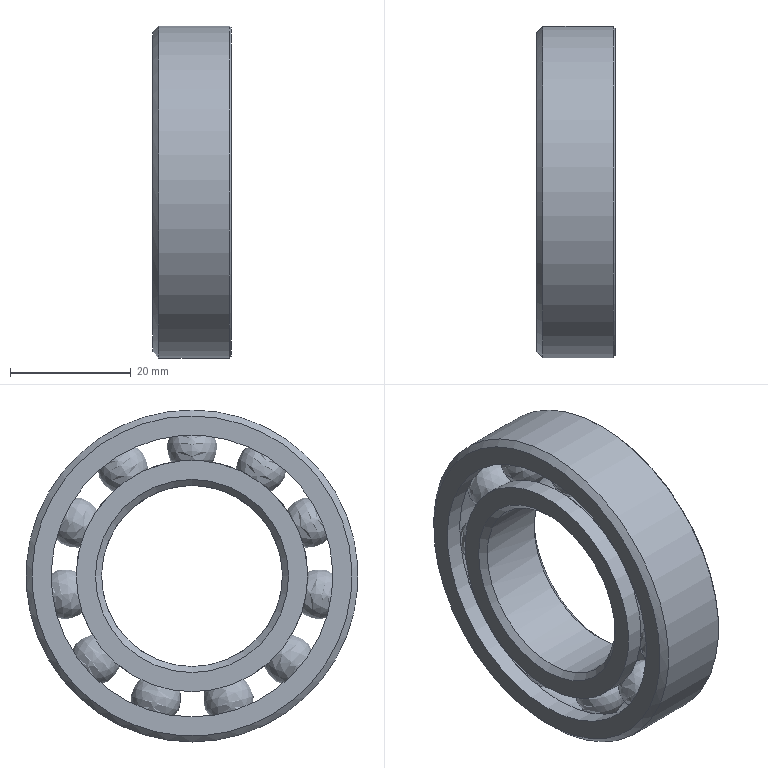Component | NX | GB-T292_AC-1994_7006_AC_3 | 13 solids | 27 faces | volume 14582 mm3 | sphere 11 | cylinder 5 | cone 5 | plane 4 | torus 2 | commonest cylinder face diameters 38.334 x2 30 x1 55 x1 46.666 x1